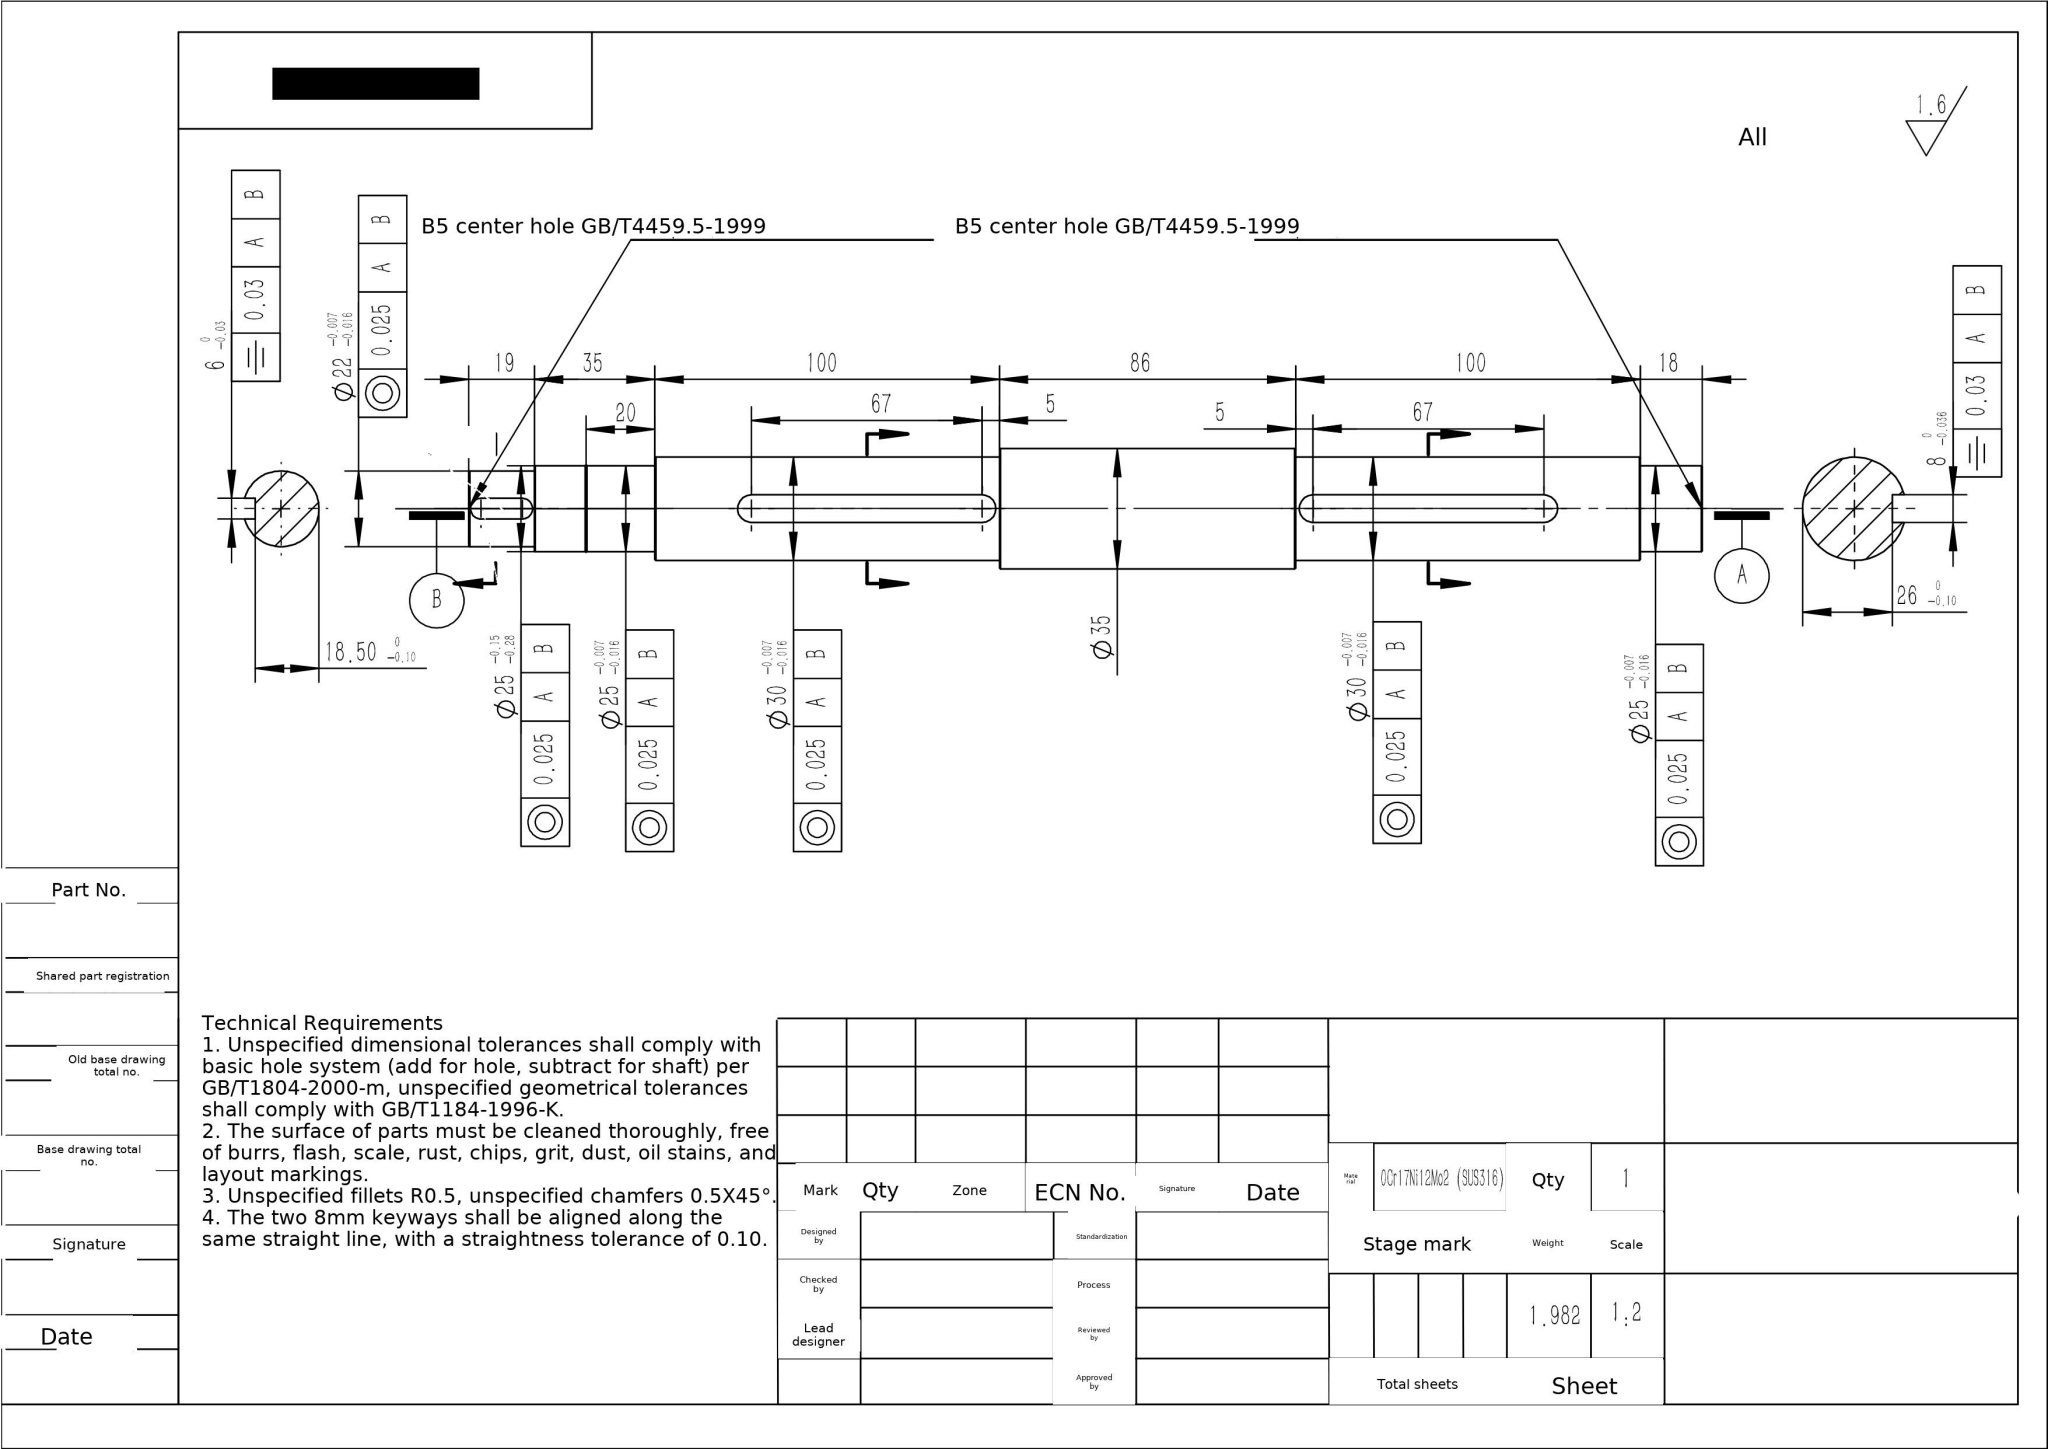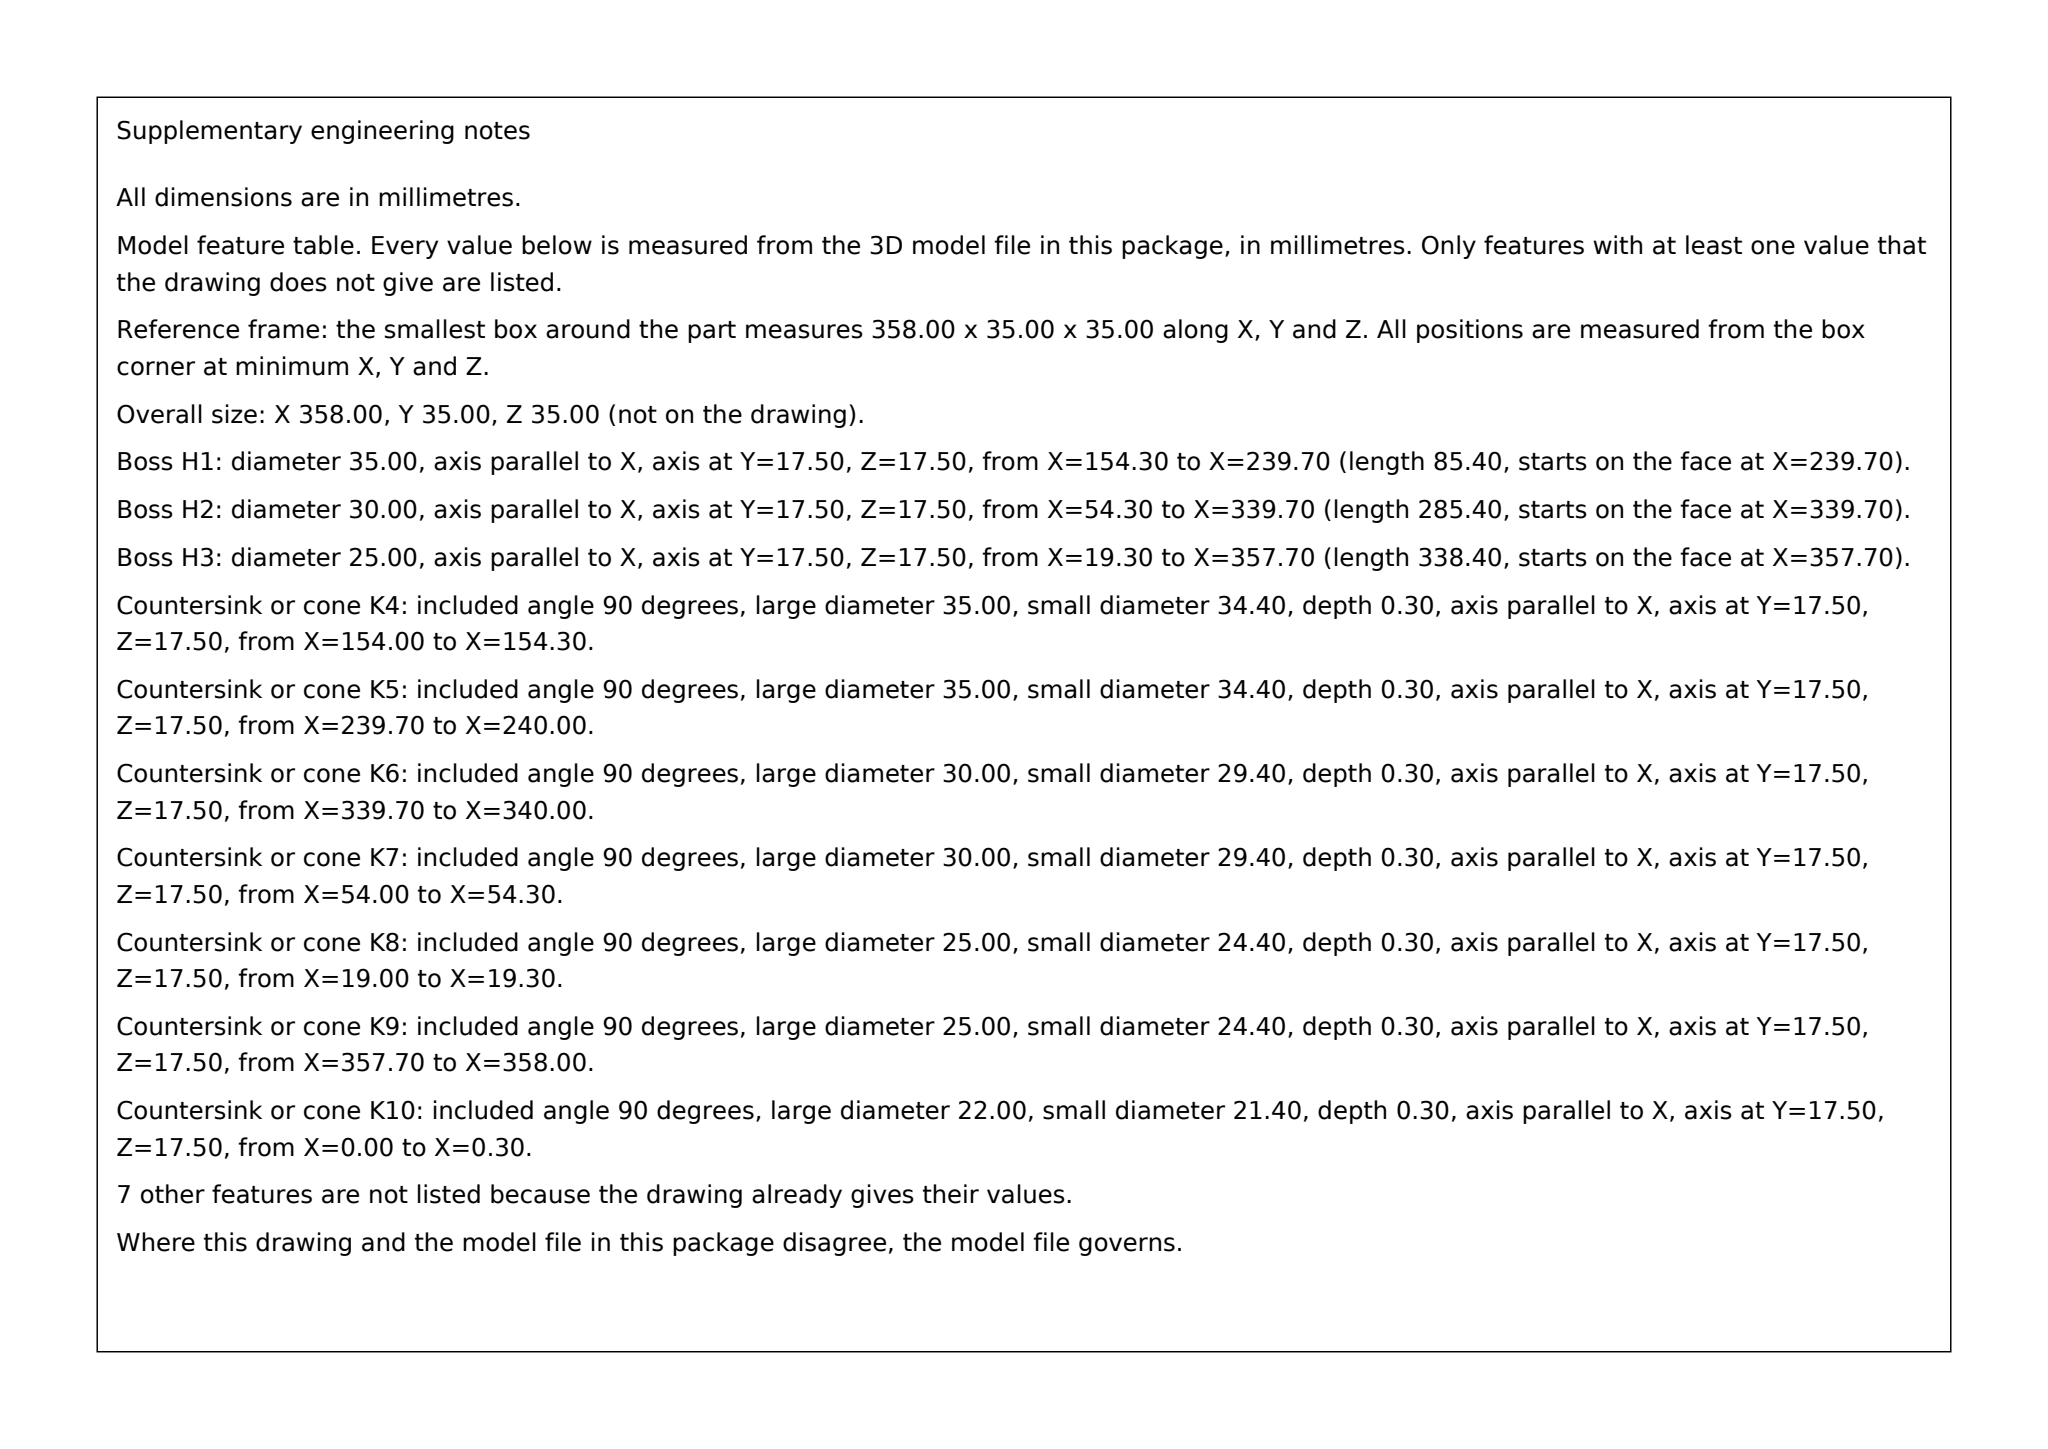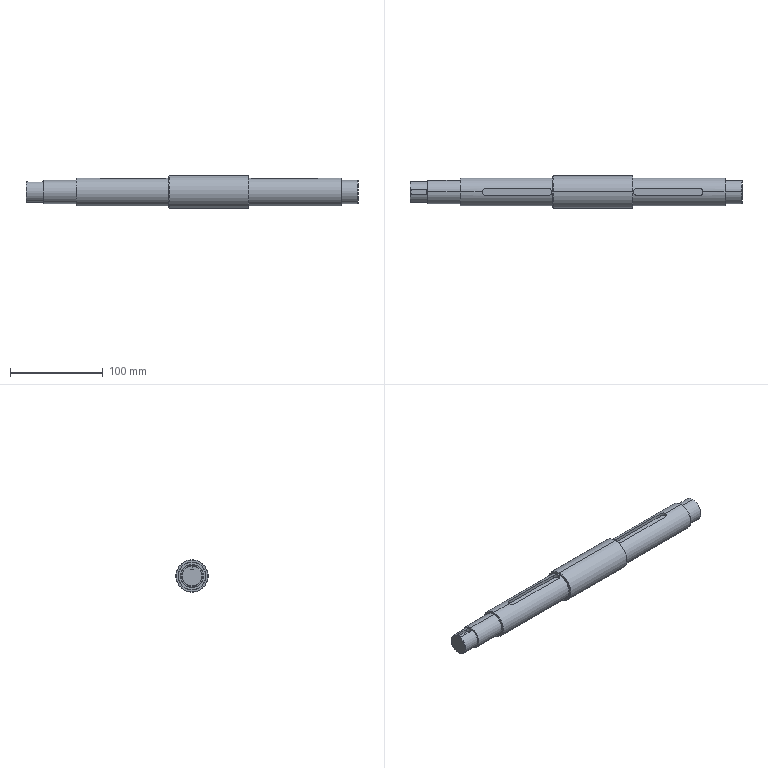Part | SolidWorks | mm | material 0Cr17Ni12Mo2 (SUS316) | 1 solid | 51 faces | box 358 x 35 x 35 mm | volume 252502 mm3 | cylinder 21 | plane 16 | cone 14 | commonest cylinder face diameters 8 x6 25 x4 30 x4 6 x3 35 x2 22 x2
build123d program:
from build123d import *

# Parameters (mm, degrees)
CUT_EXTRUDE1_DEPTH = 10
CHAMFER1_SIZE      = 0.3
CUT_EXTRUDE2_DEPTH = 10


with BuildPart() as part:
    # Sketch1 → Revolve1 (revolve)
    with BuildSketch(Plane.XY, mode=Mode.PRIVATE) as revolve1_sk:
        Polygon((0, 0), (0, 11), (19, 11), (19, 12.5), (54, 12.5), (54, 15), (154, 15), (154, 17.5), (240, 17.5), (240, 15), (340, 15), (340, 12.5), (358, 12.5), (358, 0), align=None)
    revolve(revolve1_sk.sketch.rotate(Axis((0, 0, 0), (1, 0, 0)), 90), axis=Axis((0, 0, 0), (1, 0, 0)))

    # Sketch2 → Cut-Extrude1 (cut)
    with BuildSketch(Plane.XY.offset(11)):
        with BuildLine():
            Line((149, -4), (82, -4))
            ThreePointArc((82, -4), (78, 0), (82, 4))
            Line((82, 4), (149, 4))
            ThreePointArc((149, 4), (153, 0), (149, -4))
        make_face()
        with BuildLine():
            Line((312, -4), (245, -4))
            ThreePointArc((245, -4), (241, 0), (245, 4))
            Line((245, 4), (312, 4))
            ThreePointArc((312, 4), (316, 0), (312, -4))
        make_face()
    extrude(amount=CUT_EXTRUDE1_DEPTH, mode=Mode.SUBTRACT)

    # Chamfer1
    chamfer1_edges = [part.edges().sort_by_distance(p)[0] for p in [
        (340, 0, -15),
        (240, 0, -17.5),
        (154, 0, -17.5),
        (54, 0, -15),
        (19, 0, -12.5),
        (0, 0, -11),
        (358, 0, -12.5),
    ]]
    chamfer(chamfer1_edges, length=CHAMFER1_SIZE)

    # Sketch5 → Cut-Extrude2 (cut)
    with BuildSketch(Plane.XY.offset(7.5)):
        with BuildLine():
            Line((15.5, -3), (3.5, -3))
            ThreePointArc((3.5, -3), (0.5, 0), (3.5, 3))
            Line((3.5, 3), (15.5, 3))
            ThreePointArc((15.5, 3), (18.5, 0), (15.5, -3))
        make_face()
    extrude(amount=CUT_EXTRUDE2_DEPTH, mode=Mode.SUBTRACT)


solid = part.part